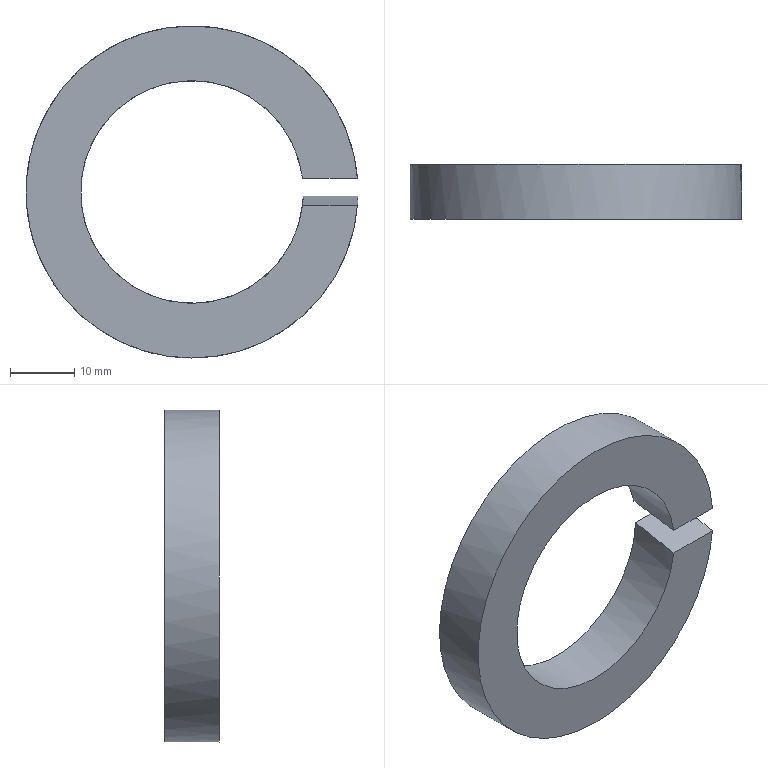Component | NX | GB93-87__33 | 1 solid | 6 faces | volume 9493 mm3 | plane 4 | cylinder 2 | commonest cylinder face diameters 51.7 x1 34.7 x1